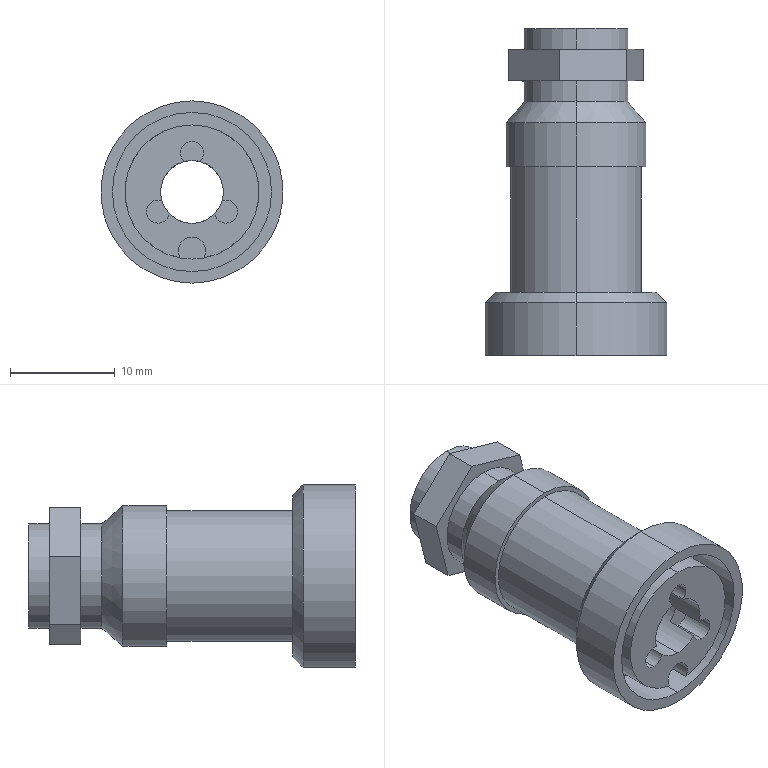Component | SolidWorks | AviationExternalConnector-1 | 1 solid | 46 faces | box 17.4 x 31.2 x 17.4 mm | volume 3142 mm3 | cylinder 24 | plane 18 | cone 4 | commonest cylinder face diameters 2.2 x7 10 x4 12.8 x2 15.2 x2 6 x2 17.4 x2 12.5 x2 13.4 x2
build123d program:
from build123d import *

# Parameters (mm, degrees)
BOSS_EXTRUDE1_DEPTH           = 3
SKETCH3_R                     = 3
CUT_EXTRUDE1_DEPTH            = 34.538
CHAMFER1_SIZE                 = 1
SOCKETSLEEVERELIEF_SKETCH_R   = 7.6
SOCKETSLEEVERELIEF_SKETCH_R_2 = 6.4
SOCKETSLEEVERELIEF_DEPTH      = 5.2
SOCKETPINKEYRELIEF_SKETCH_R   = 1.1
SOCKETPINKEYRELIEF_SKETCH_R_2 = 1.3
SOCKETPINKEYRELIEF_DEPTH      = 3.2


with BuildPart() as part:
    # Sketch1 → Revolve1 (revolve)
    with BuildSketch(Plane.XY, mode=Mode.PRIVATE) as revolve1_sk:
        Polygon((0, 0), (5, 0), (5, -7), (6.7, -9), (6.7, -13.2), (6.25, -13.2), (6.25, -25.2), (8.7, -25.2), (8.7, -31.2), (0, -31.2), align=None)
    revolve(revolve1_sk.sketch.rotate(Axis((0, 0, 0), (0, -1, 0)), 90), axis=Axis((0, 0, 0), (0, -1, 0)))

    # Sketch2 → Boss-Extrude1 (add)
    with BuildSketch(Plane(origin=(0, -2, 0), x_dir=(1, 0, 0), z_dir=(0, 1, 0))):
        Polygon((-1.6, -6.506), (4.834, -4.639), (6.435, 1.867), (1.6, 6.506), (-4.834, 4.639), (-6.435, -1.867), align=None)
    extrude(amount=-BOSS_EXTRUDE1_DEPTH)

    # Sketch3 → Cut-Extrude1 (cut, through all)
    with BuildSketch(Plane(origin=(0, 0, 0), x_dir=(1, 0, 0), z_dir=(0, 1, 0))):
        with Locations(Location((0, 0, 0), (0, 0, 270))):
            Circle(SKETCH3_R)
    extrude(amount=-CUT_EXTRUDE1_DEPTH, mode=Mode.SUBTRACT)

    # Chamfer1
    chamfer1_edges = [part.edges().sort_by_distance(p)[0] for p in [
        (0, -25.2, -8.7),
    ]]
    chamfer(chamfer1_edges, length=CHAMFER1_SIZE)

    # SocketSleeveRelief_Sketch → SocketSleeveRelief (cut)
    with BuildSketch(Plane.XZ.offset(31.2)):
        with Locations(Location((0, 0, 0), (0, 0, 270))):
            Circle(SOCKETSLEEVERELIEF_SKETCH_R)
        with Locations(Location((0, 0, 0), (0, 0, 270))):
            Circle(SOCKETSLEEVERELIEF_SKETCH_R_2, mode=Mode.SUBTRACT)
    extrude(amount=-SOCKETSLEEVERELIEF_DEPTH, mode=Mode.SUBTRACT)

    # SocketPinKeyRelief_Sketch → SocketPinKeyRelief (cut)
    with BuildSketch(Plane.XZ.offset(31.2)):
        with Locations((0, 3.75)):
            Circle(SOCKETPINKEYRELIEF_SKETCH_R)
        with Locations((3.248, -1.875)):
            Circle(SOCKETPINKEYRELIEF_SKETCH_R)
        with Locations((-3.248, -1.875)):
            Circle(SOCKETPINKEYRELIEF_SKETCH_R)
        with Locations((0, -5.6)):
            Circle(SOCKETPINKEYRELIEF_SKETCH_R_2)
    extrude(amount=-SOCKETPINKEYRELIEF_DEPTH, mode=Mode.SUBTRACT)


solid = part.part

# Placed as in the assembly
solid = solid.moved(Location((1197.686, 1596.512, 2265.983), (0, 0, 0)))